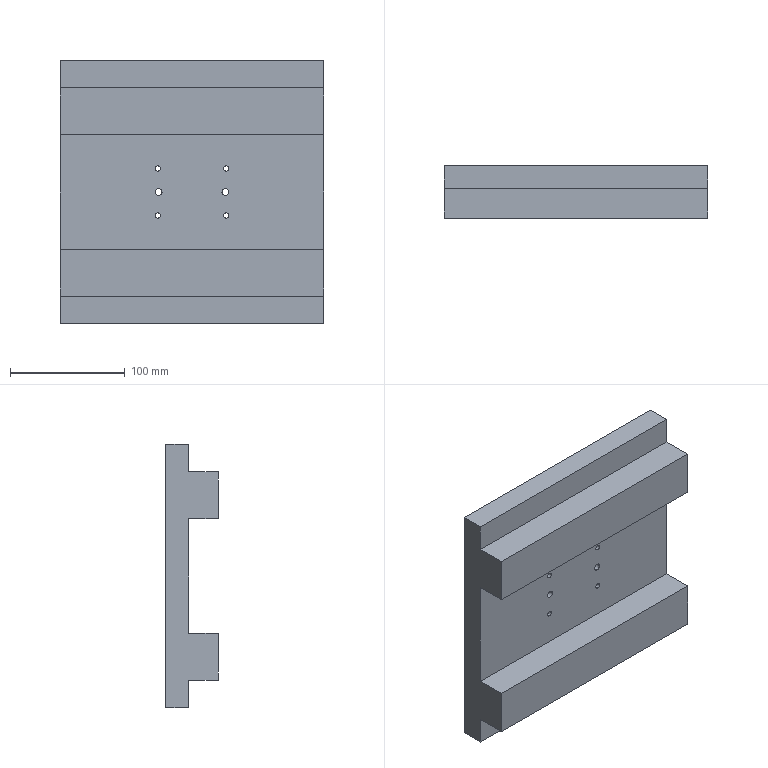Component | SolidWorks | WorkPlatform-1 | 1 solid | 41 faces | box 230 x 46 x 230 mm | volume 1541443 mm3 | cylinder 22 | plane 19 | commonest cylinder face diameters 4.542 x8 8.034 x8 5.965 x4 16.633 x2
build123d program:
from build123d import *

# Parameters (mm, degrees)
SKETCH1_W           = 230
SKETCH1_H           = 230
BOSS_EXTRUDE1_DEPTH = 20
SKETCH3_R           = 4.017
CUT_EXTRUDE1_DEPTH  = 10
SKETCH4_R           = 2.271
CUT_EXTRUDE2_DEPTH  = 48
SKETCH5_R           = 2.983
CUT_EXTRUDE3_DEPTH  = 29
SKETCH6_W           = 40.761
SKETCH6_H           = 230
BOSS_EXTRUDE2_DEPTH = 26.003
SKETCH7_R           = 8.316
CUT_EXTRUDE4_DEPTH  = 1.5


with BuildPart() as part:
    # Sketch1 → Boss-Extrude1 (new body)
    with BuildSketch(Plane(origin=(0, 0, 0), x_dir=(1, 0, 0), z_dir=(0, 1, 0))):
        Rectangle(SKETCH1_W, SKETCH1_H)
    extrude(amount=BOSS_EXTRUDE1_DEPTH)

    # Sketch3 → Cut-Extrude1 (cut)
    with BuildSketch(Plane(origin=(0, 20, 0), x_dir=(1, 0, 0), z_dir=(0, 1, 0))):
        with Locations(Location((20.473, 29.799, 0), (0, 0, 270))):
            Circle(SKETCH3_R)
        with Locations(Location((20.473, -29.799, 0), (0, 0, 90))):
            Circle(SKETCH3_R)
        with Locations(Location((-20.473, -29.799, 0), (0, 0, 270))):
            Circle(SKETCH3_R)
        with Locations(Location((-20.473, 29.799, 0), (0, 0, 90))):
            Circle(SKETCH3_R)
    extrude(amount=-CUT_EXTRUDE1_DEPTH, mode=Mode.SUBTRACT)

    # Sketch4 → Cut-Extrude2 (cut)
    with BuildSketch(Plane(origin=(0, 10, 0), x_dir=(1, 0, 0), z_dir=(0, 1, 0))):
        with Locations(Location((20.473, 29.799, 0), (0, 0, 270))):
            Circle(SKETCH4_R)
        with Locations(Location((20.473, -29.799, 0), (0, 0, 270))):
            Circle(SKETCH4_R)
        with Locations(Location((-20.473, -29.799, 0), (0, 0, 270))):
            Circle(SKETCH4_R)
        with Locations(Location((-20.473, 29.799, 0), (0, 0, 270))):
            Circle(SKETCH4_R)
    extrude(amount=-CUT_EXTRUDE2_DEPTH, mode=Mode.SUBTRACT)

    # Sketch5 → Cut-Extrude3 (cut)
    with BuildSketch(Plane(origin=(0, 20, 0), x_dir=(1, 0, 0), z_dir=(0, 1, 0))):
        with Locations(Location((0, 29.142, 0), (0, 0, 270))):
            Circle(SKETCH5_R)
        with Locations(Location((0, -29.142, 0), (0, 0, 270))):
            Circle(SKETCH5_R)
    extrude(amount=-CUT_EXTRUDE3_DEPTH, mode=Mode.SUBTRACT)

    # Sketch6 → Boss-Extrude2 (add)
    with BuildSketch(Plane.XZ):
        with Locations((-70.515, 0)):
            Rectangle(SKETCH6_W, SKETCH6_H)
    boss_extrude2 = extrude(amount=BOSS_EXTRUDE2_DEPTH)

    # Mirror1: Boss-Extrude2 across plane
    add(boss_extrude2.mirror(Plane.ZY))

    # Sketch7 → Cut-Extrude4 (cut)
    with BuildSketch(Plane.XY.offset(115)):
        with Locations((67.772, -0.5408)):
            Circle(SKETCH7_R)
    extrude(amount=-CUT_EXTRUDE4_DEPTH, mode=Mode.SUBTRACT)


solid = part.part

# Placed as in the assembly
solid = solid.moved(Location((56.772, 96.74, 0), (0, 90, 0)))